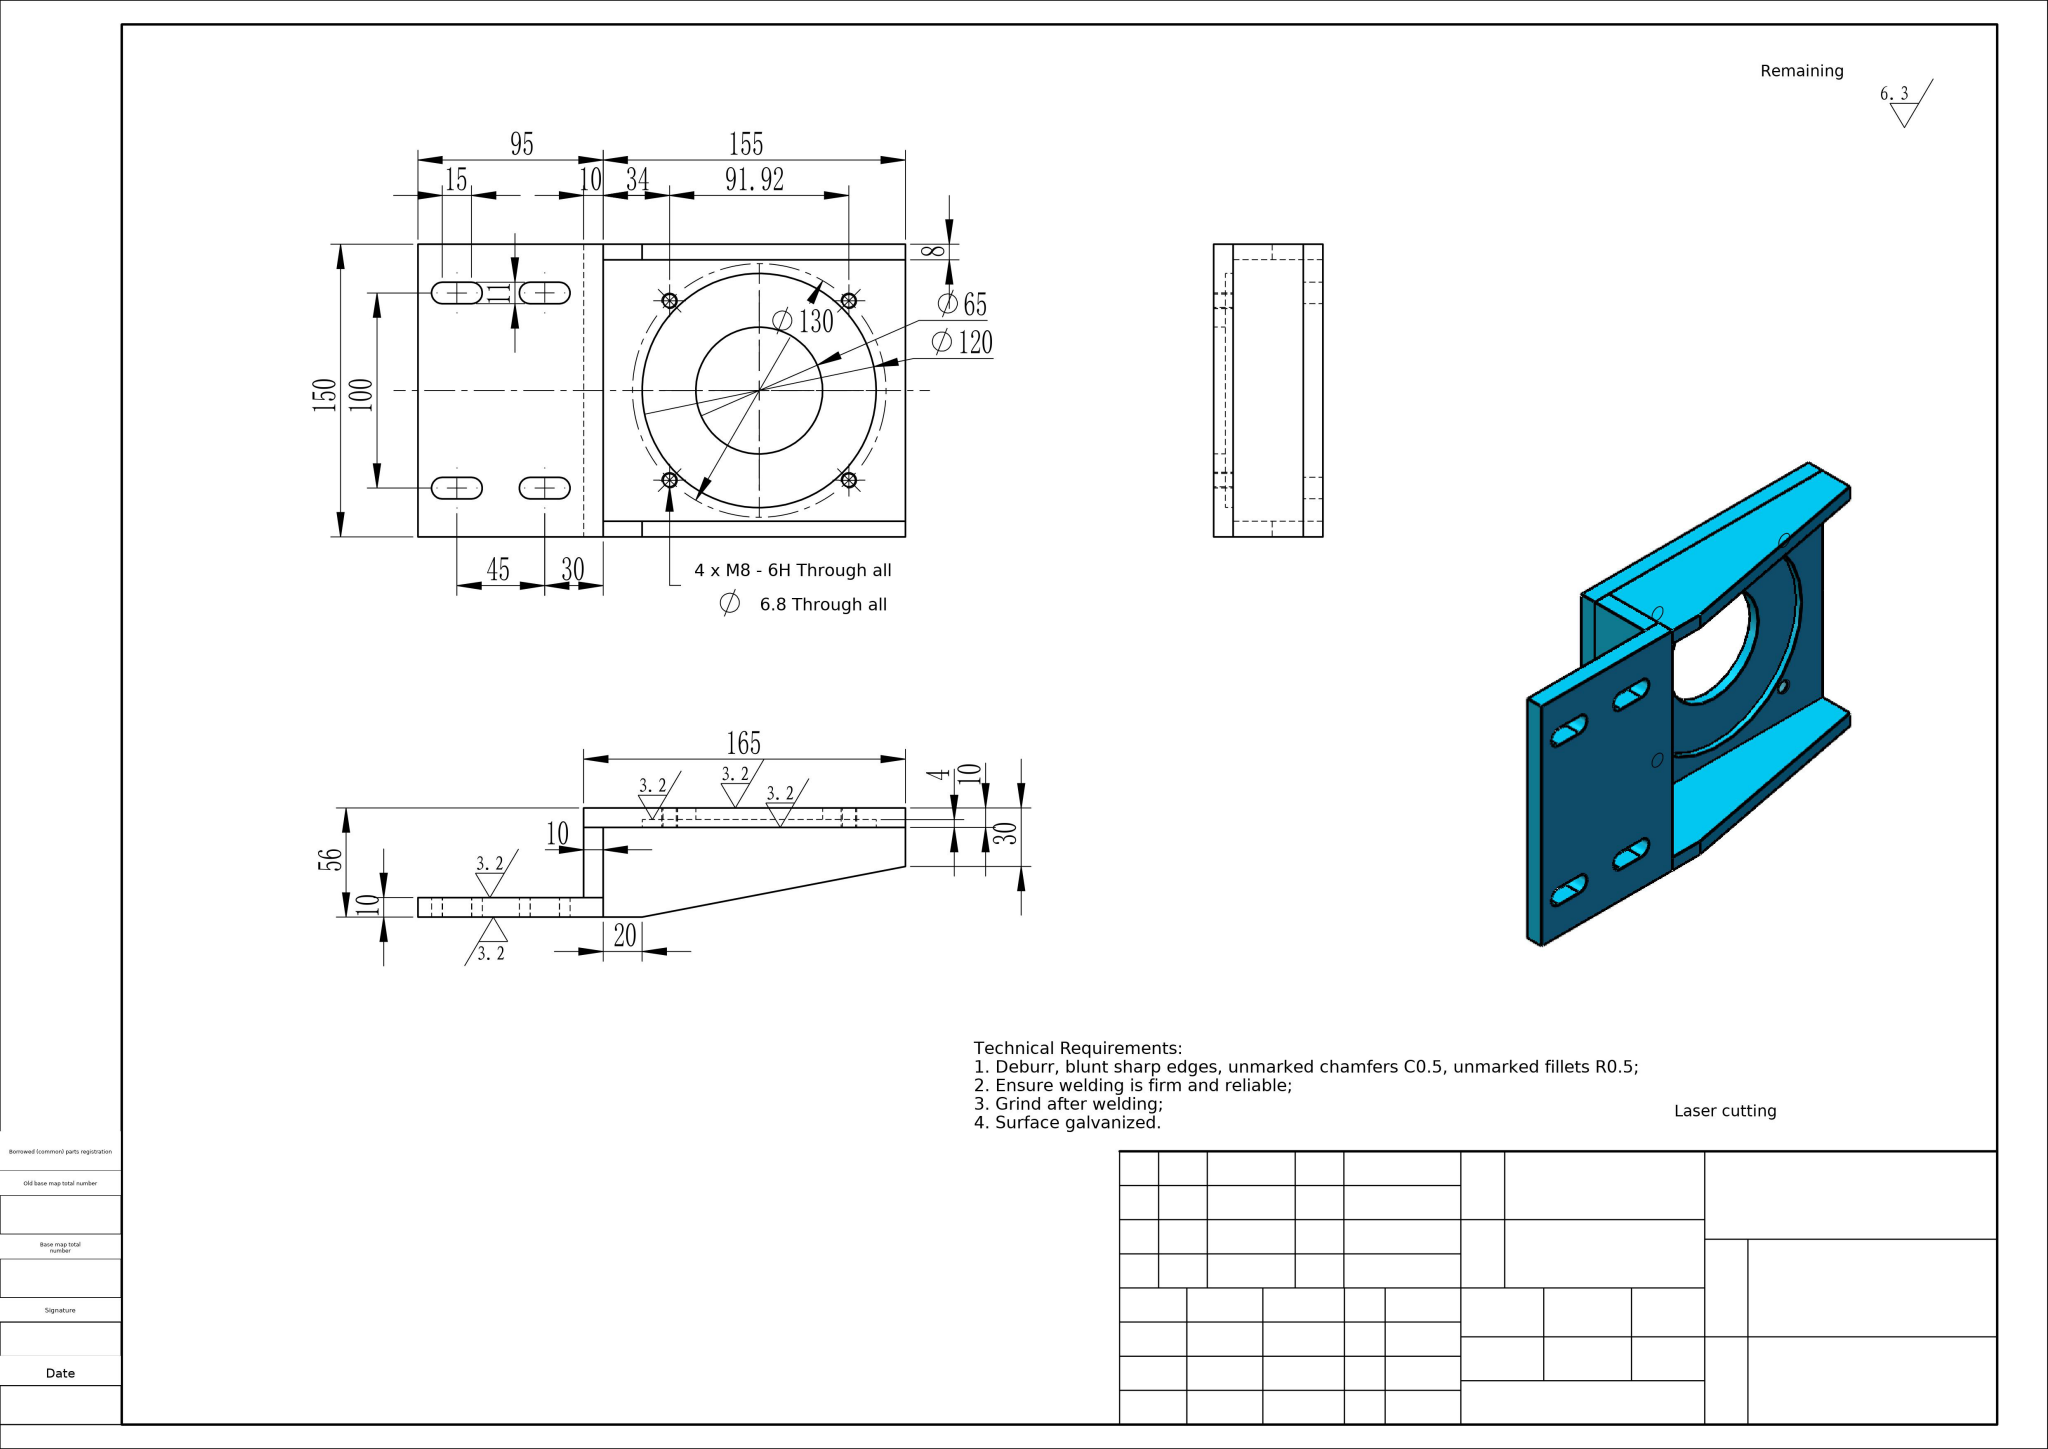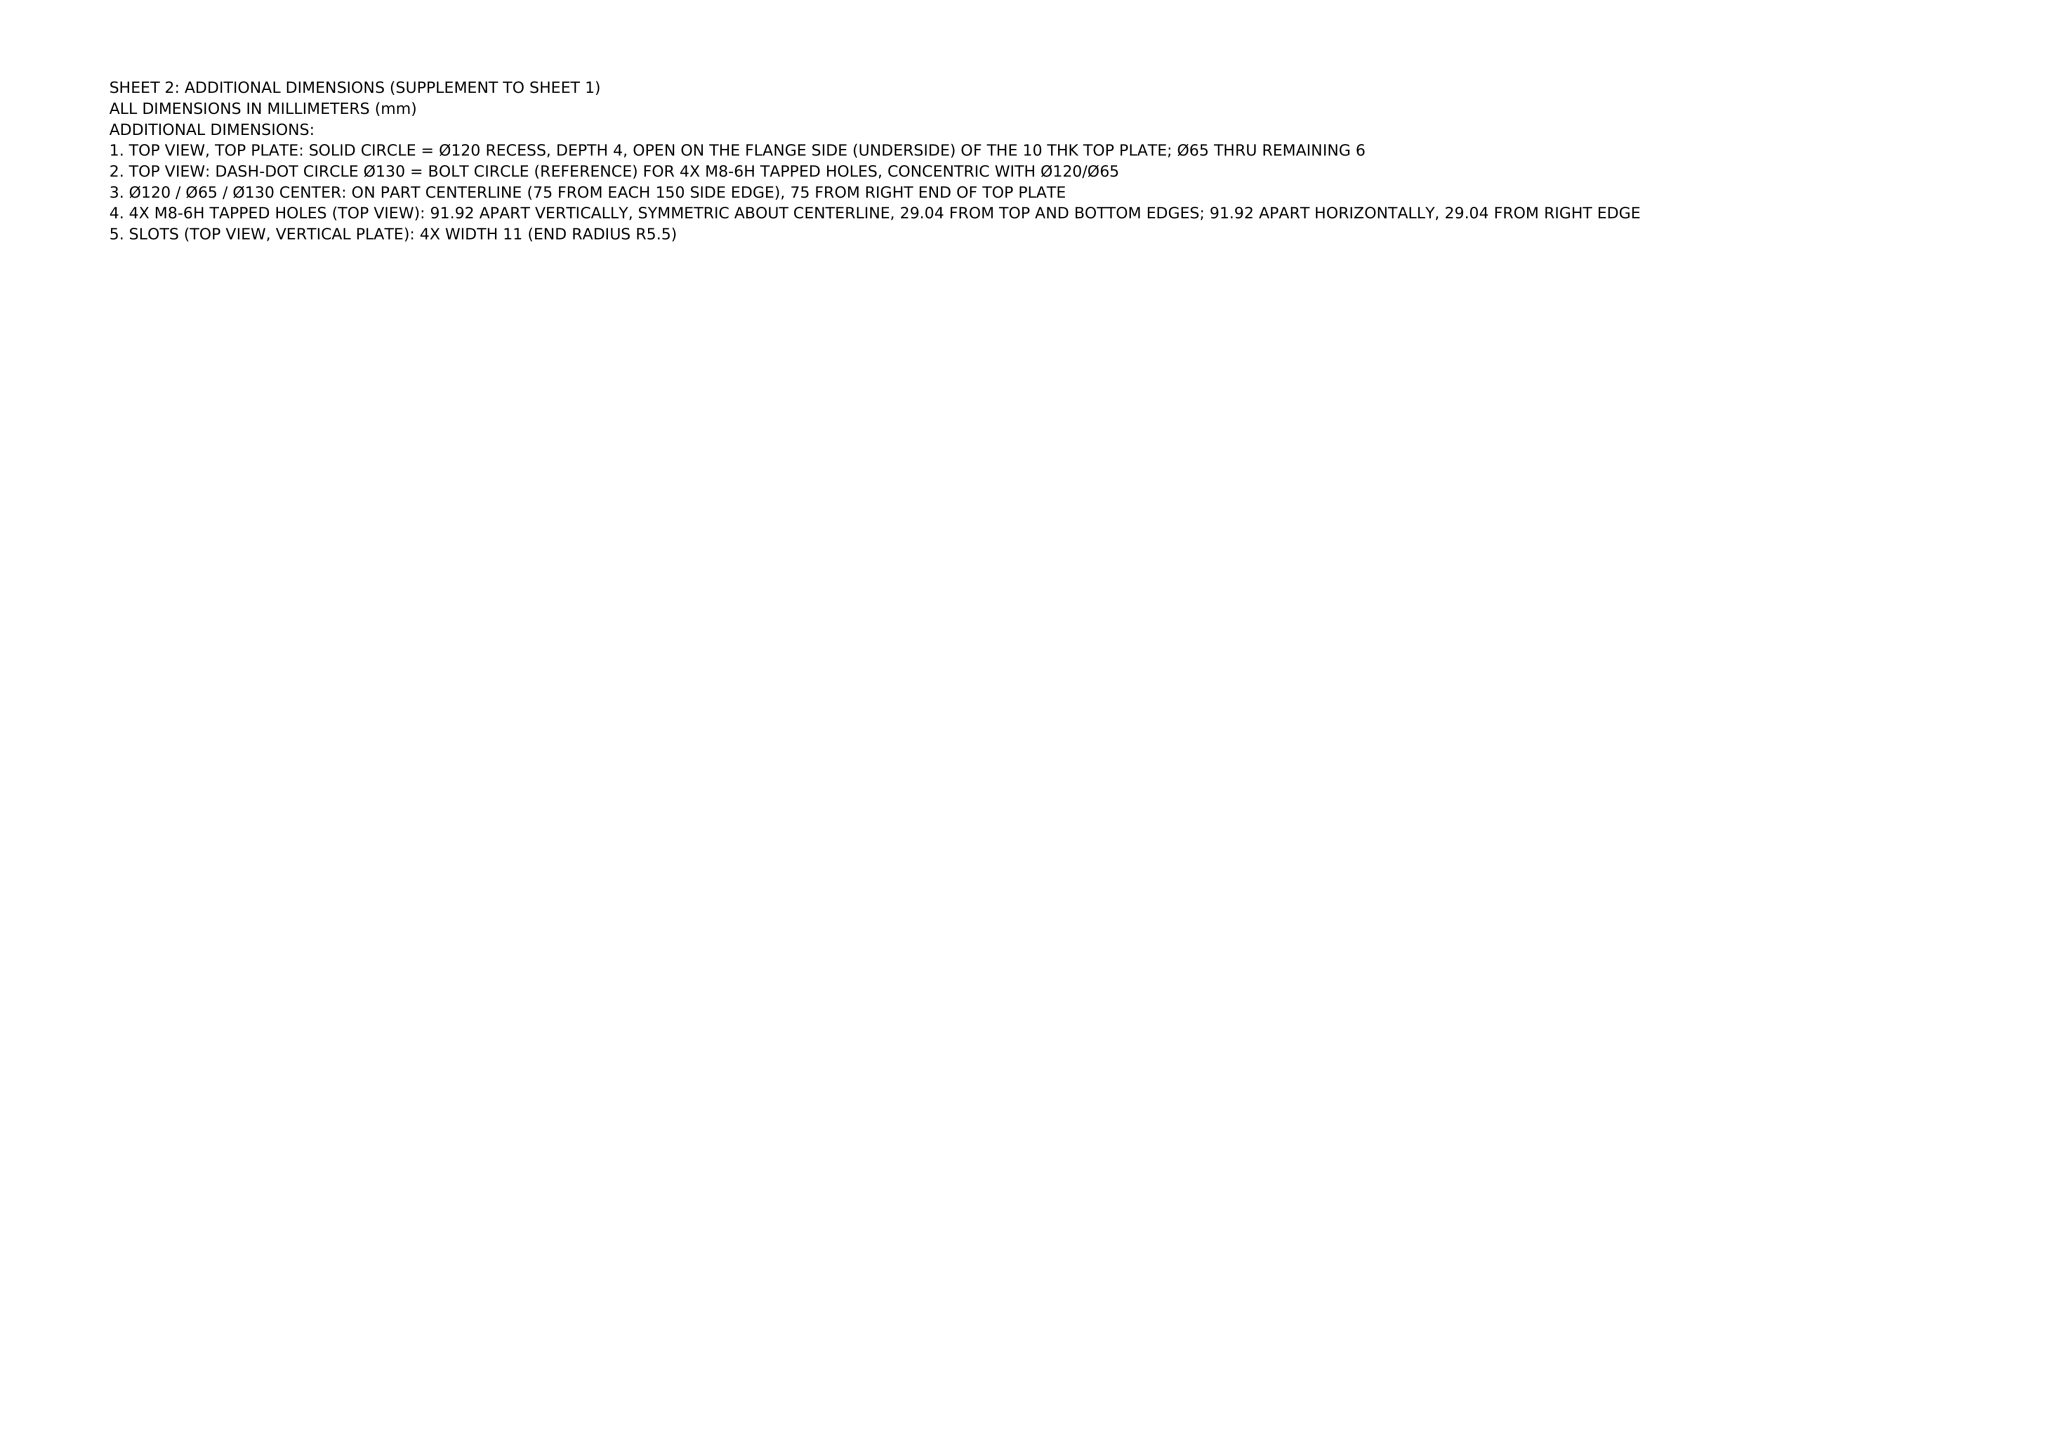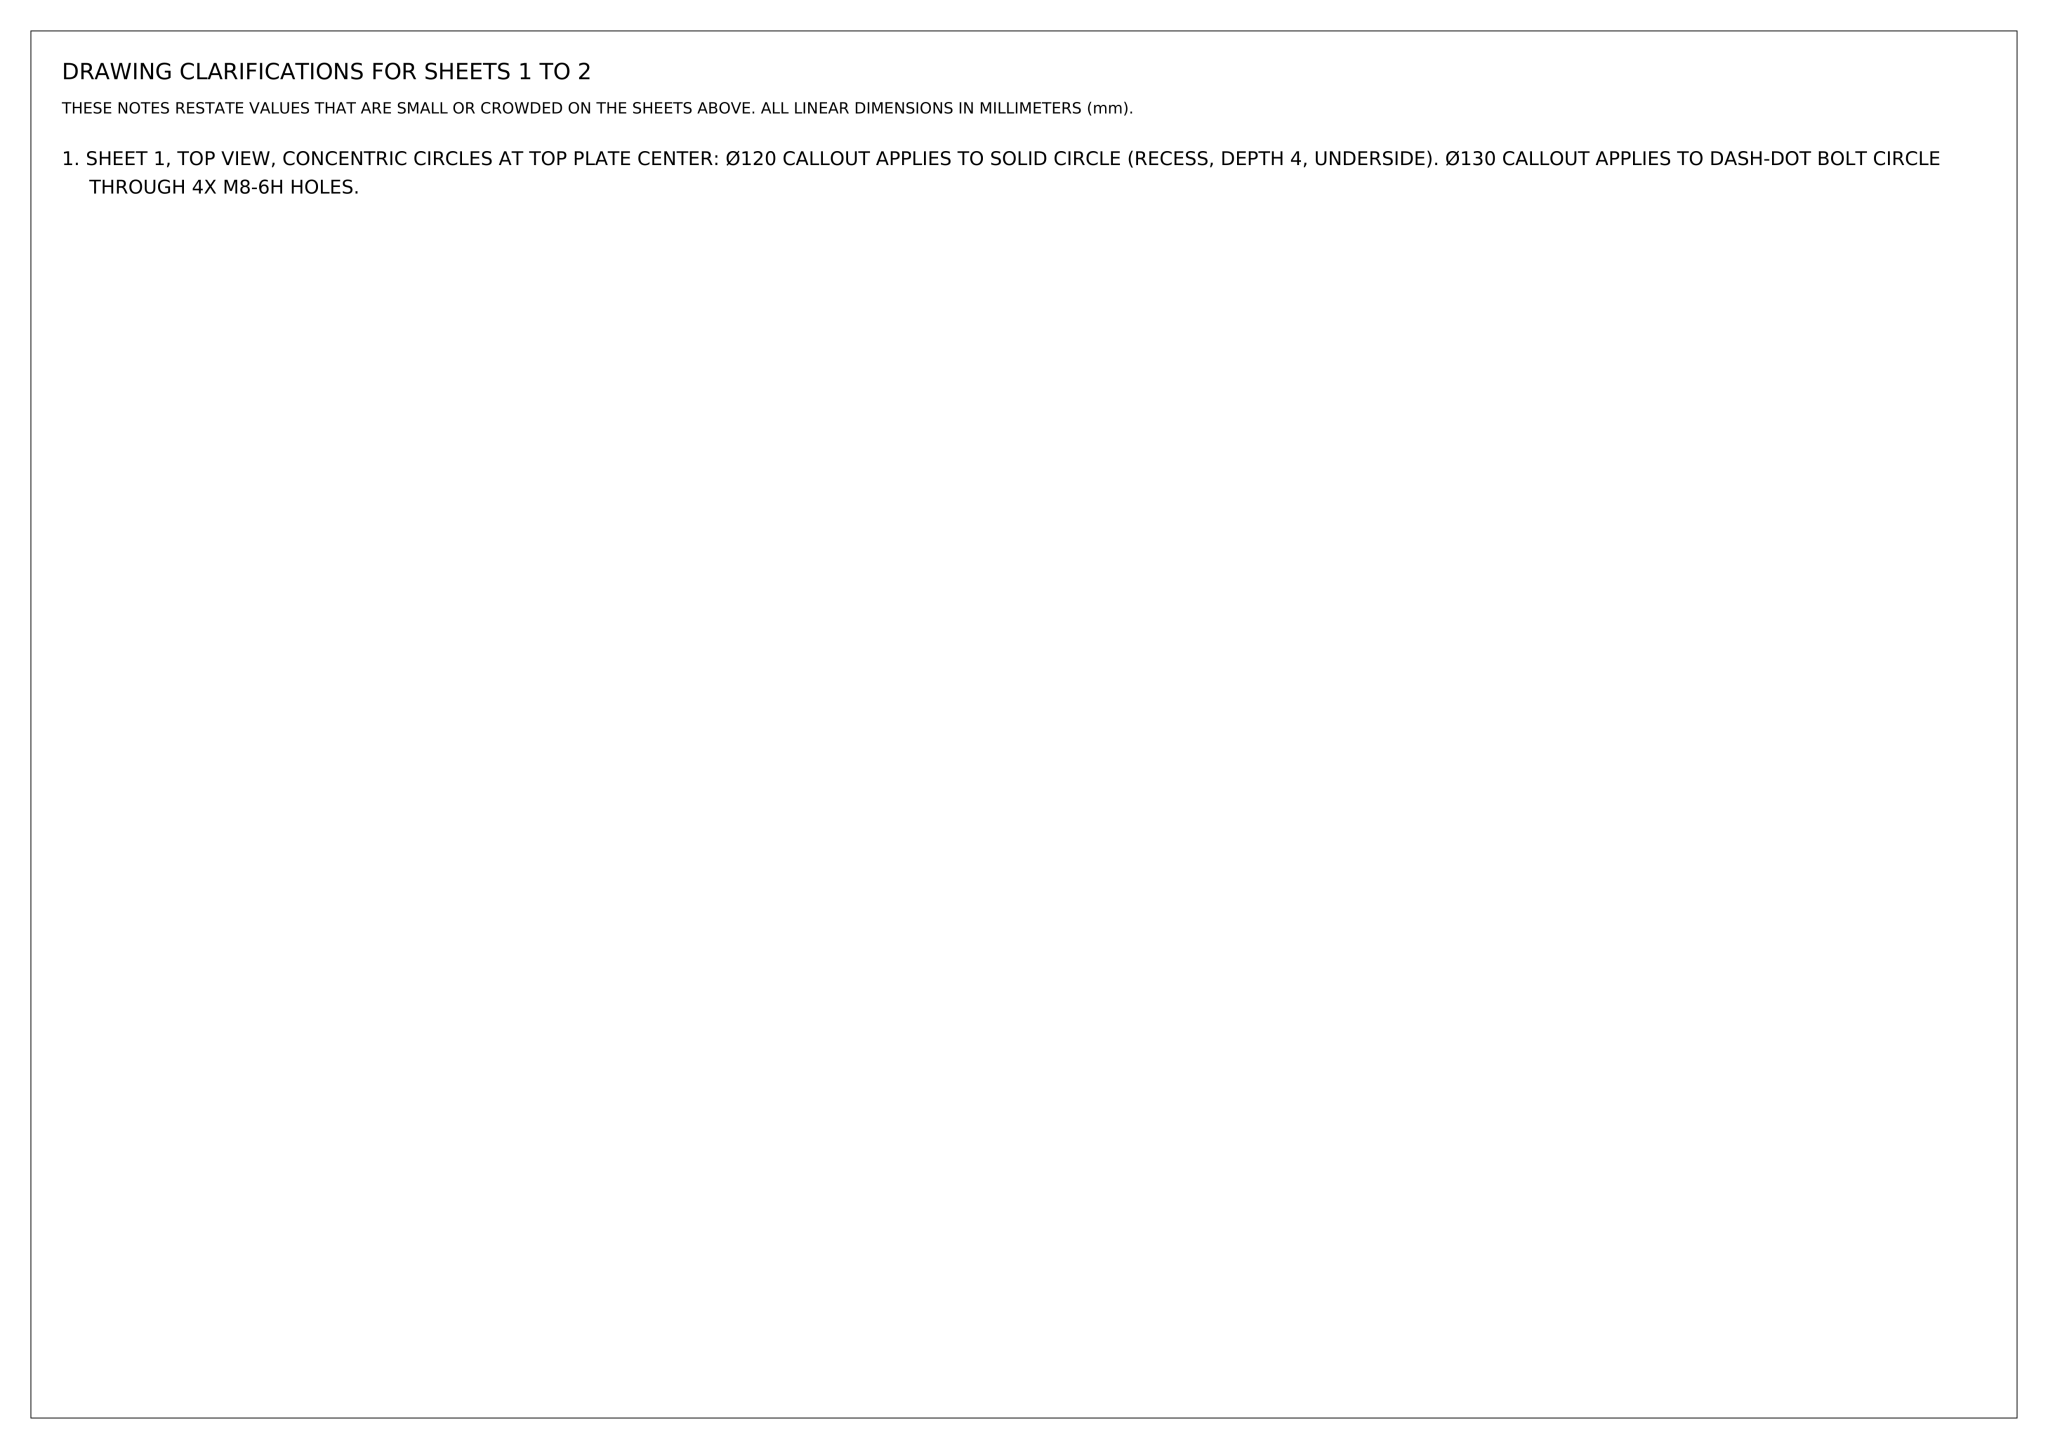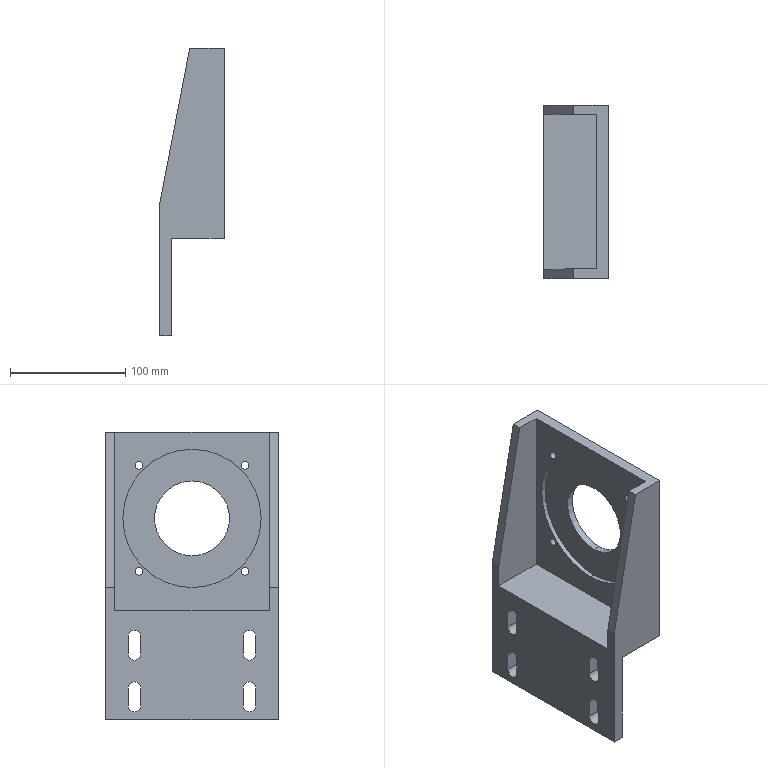Part | NX | mm | 1 solid | 47 faces | box 56 x 150 x 250 mm | volume 452997 mm3 | cylinder 24 | plane 23 | commonest cylinder face diameters 11 x12 6.8 x8 65 x2 120 x2